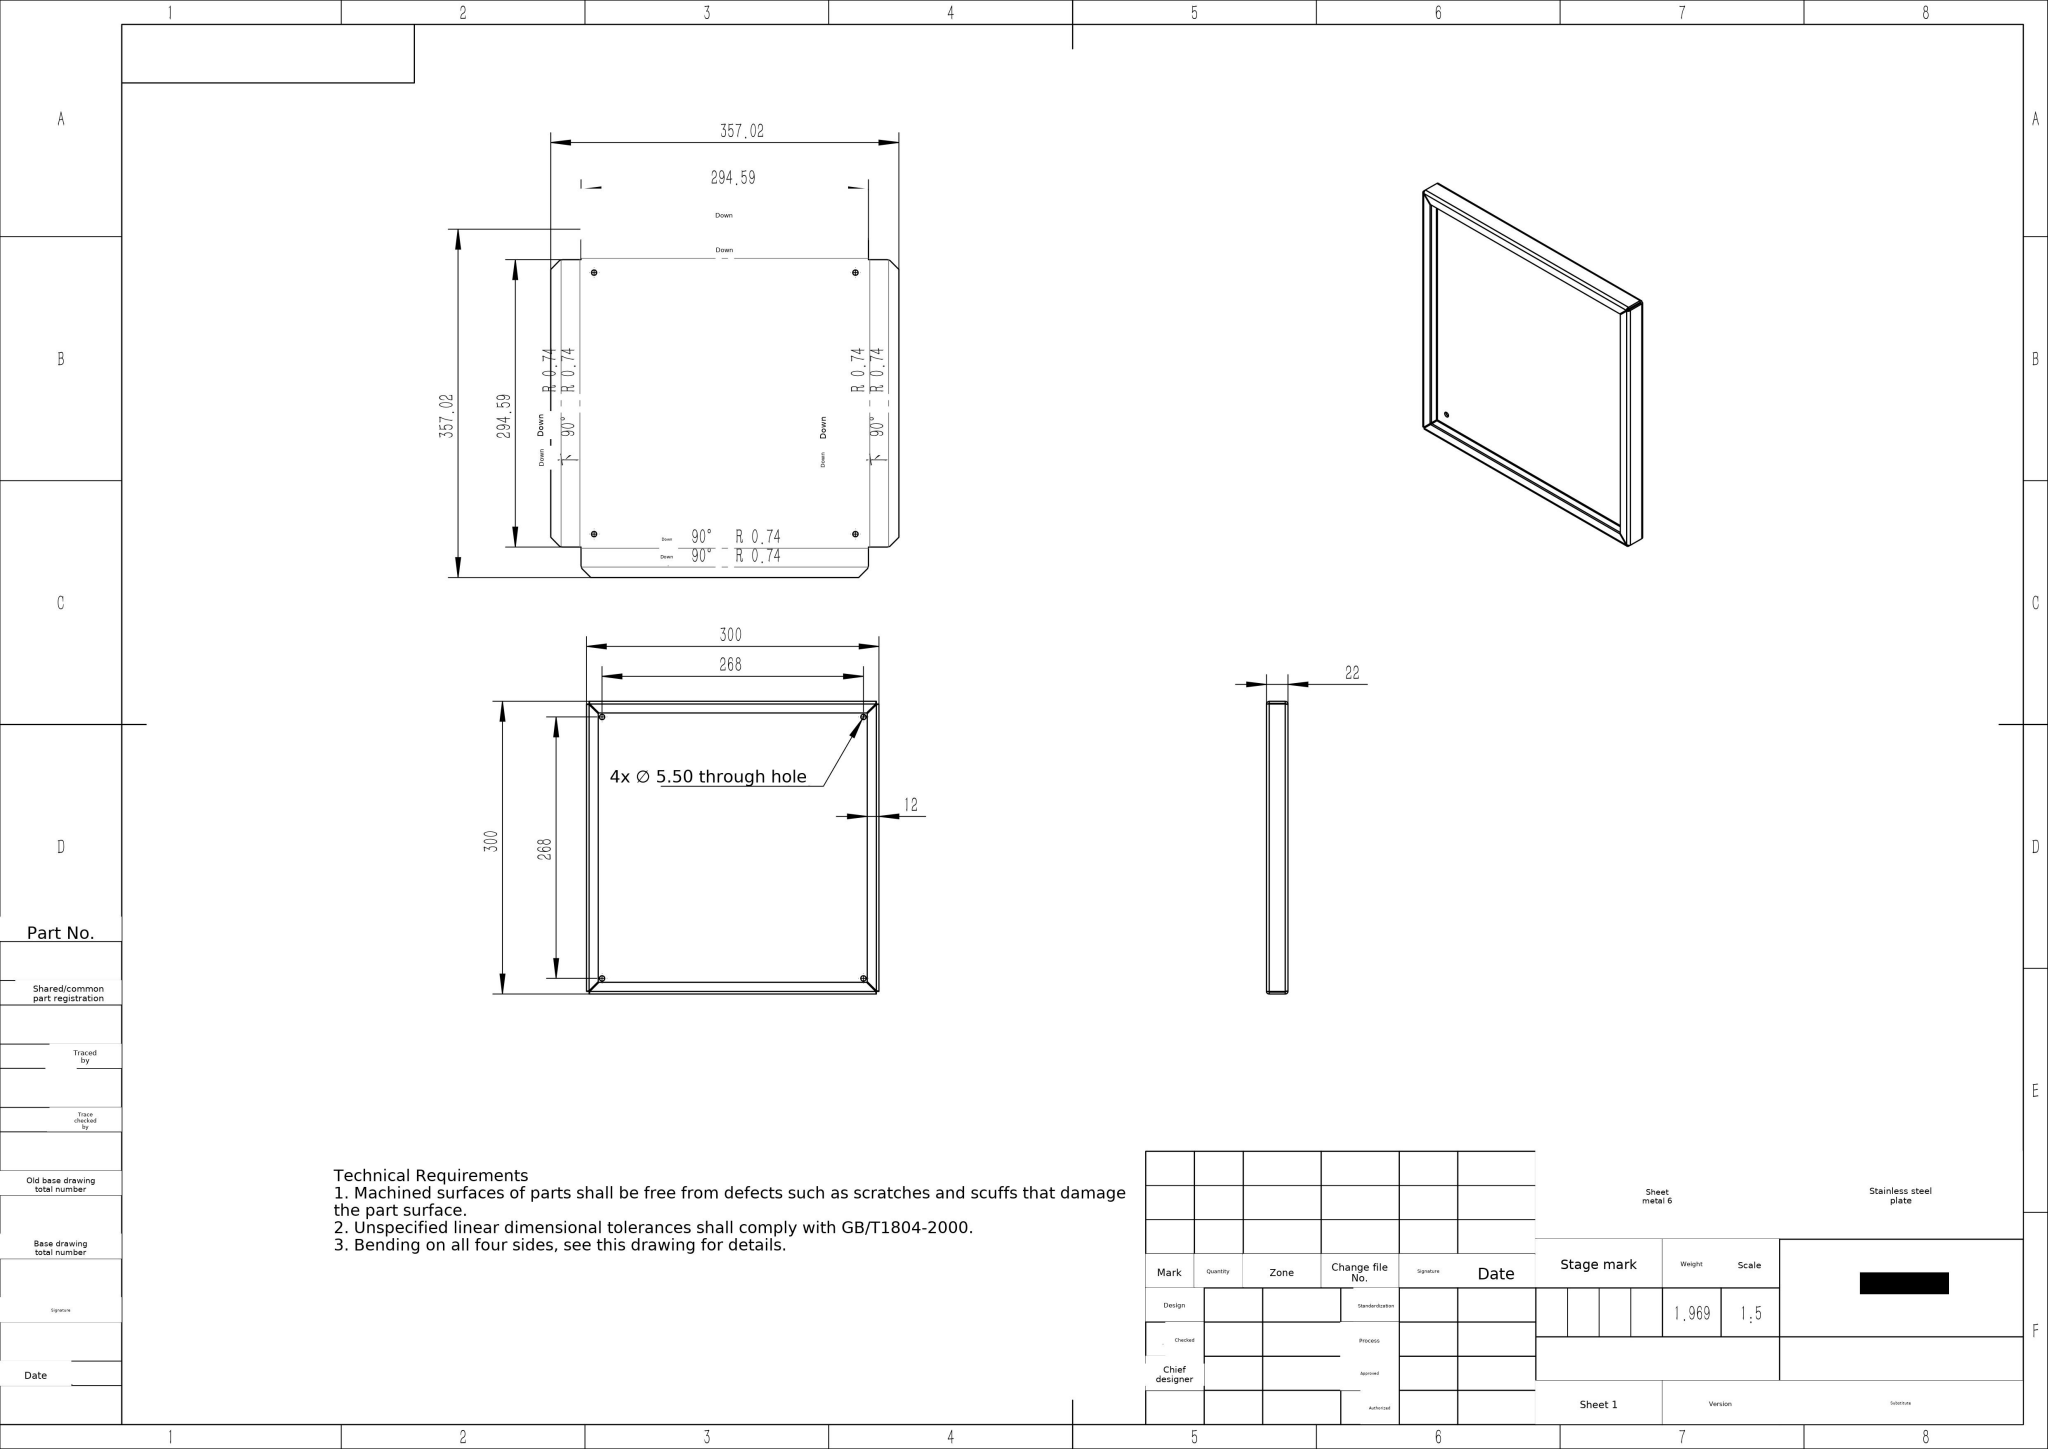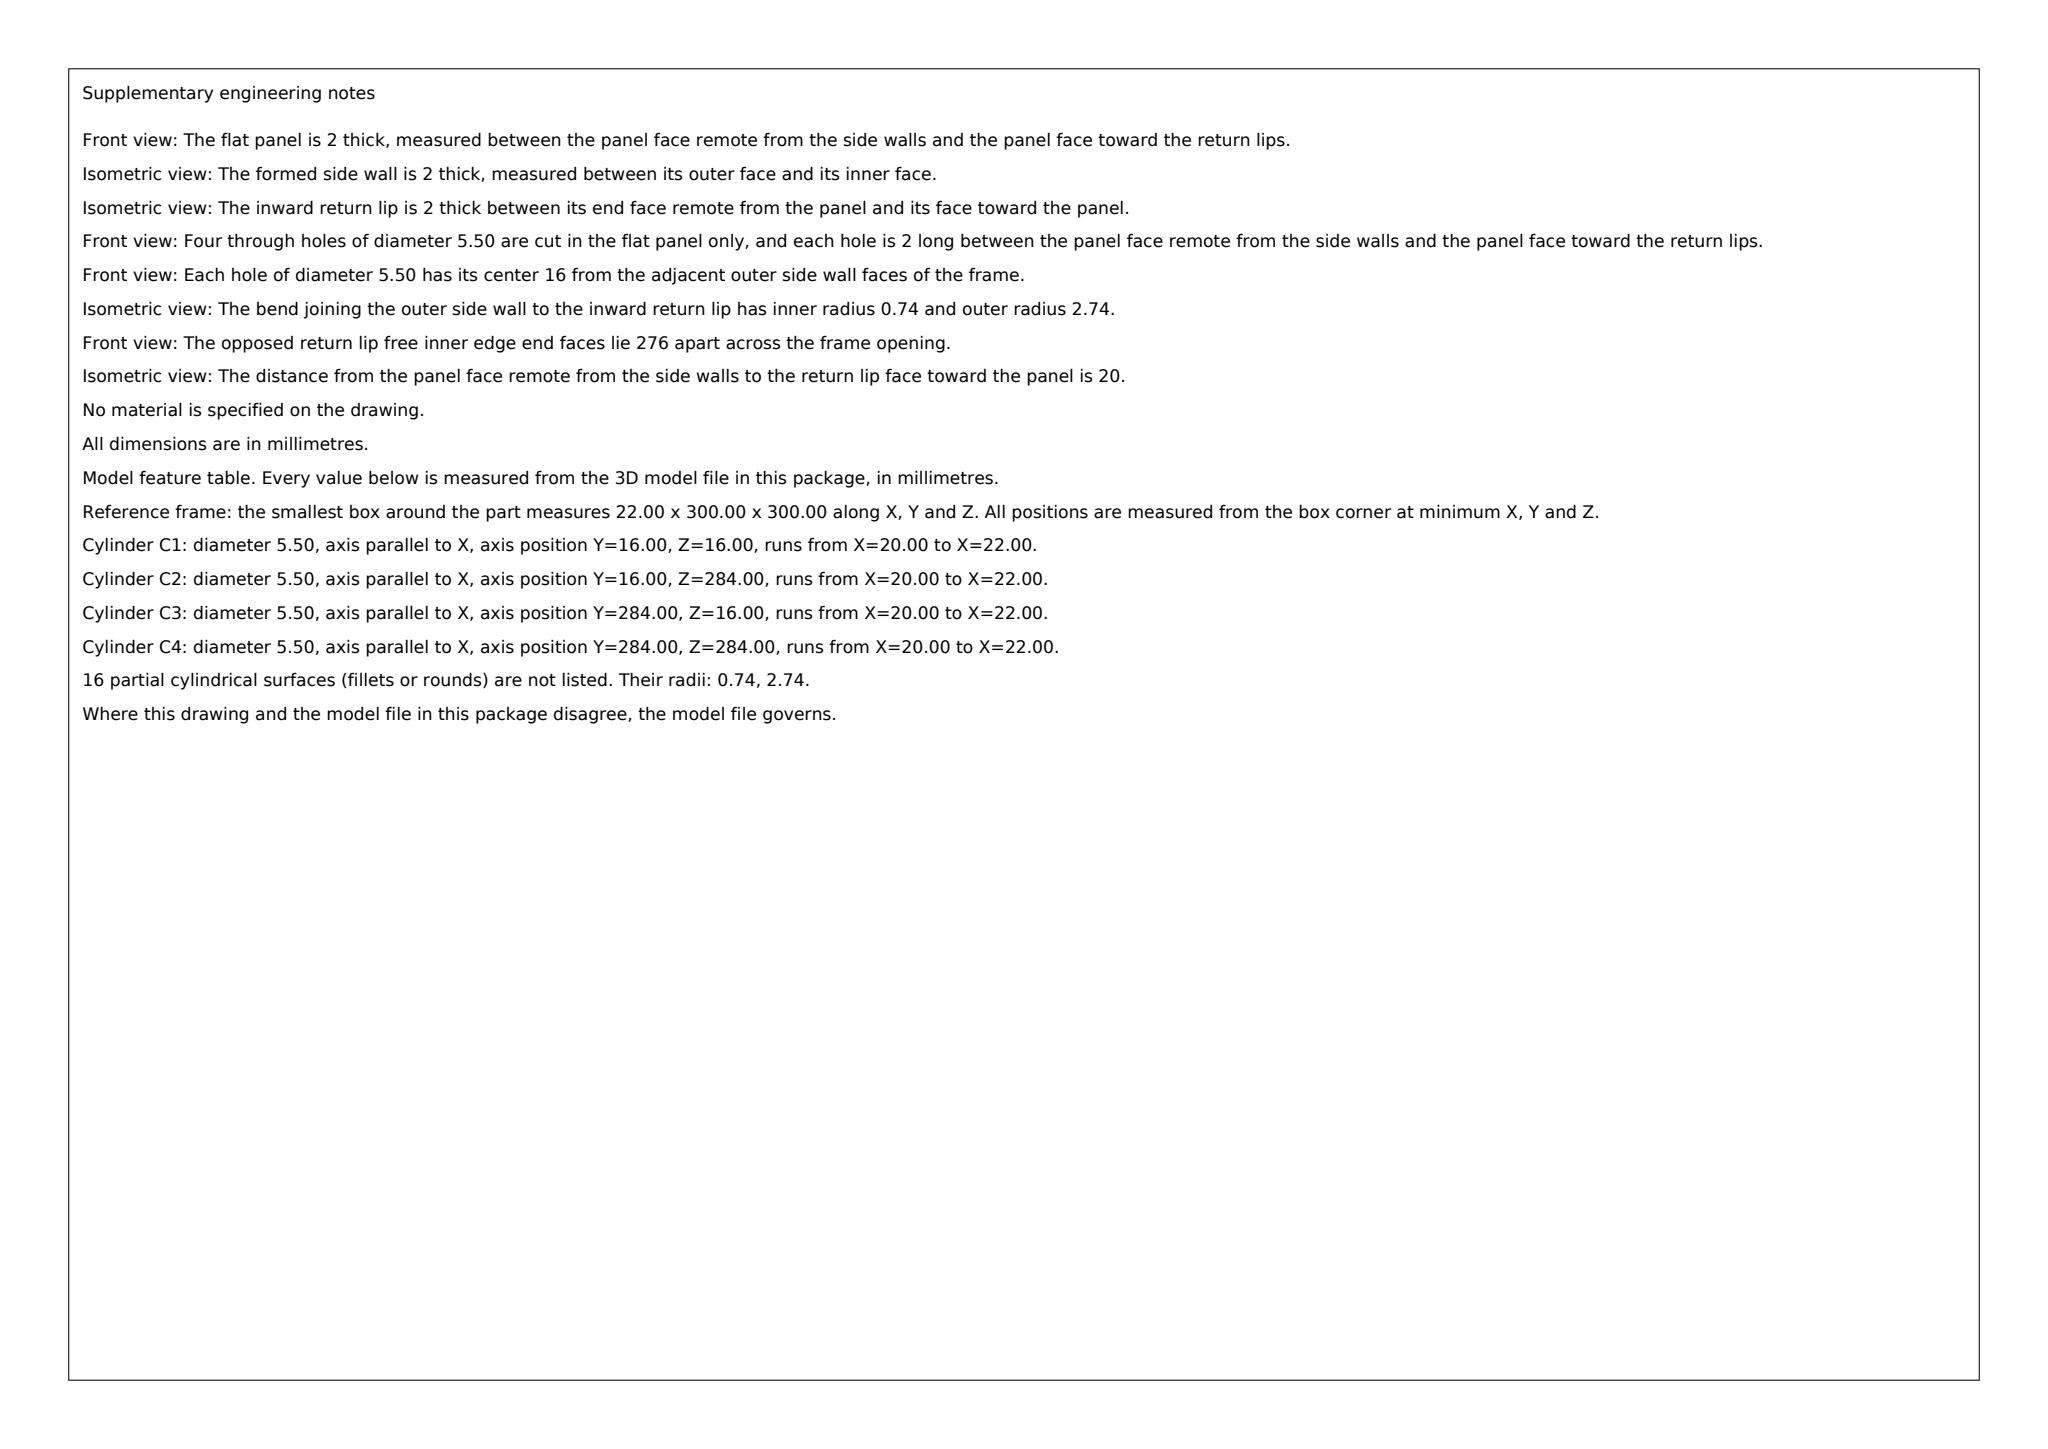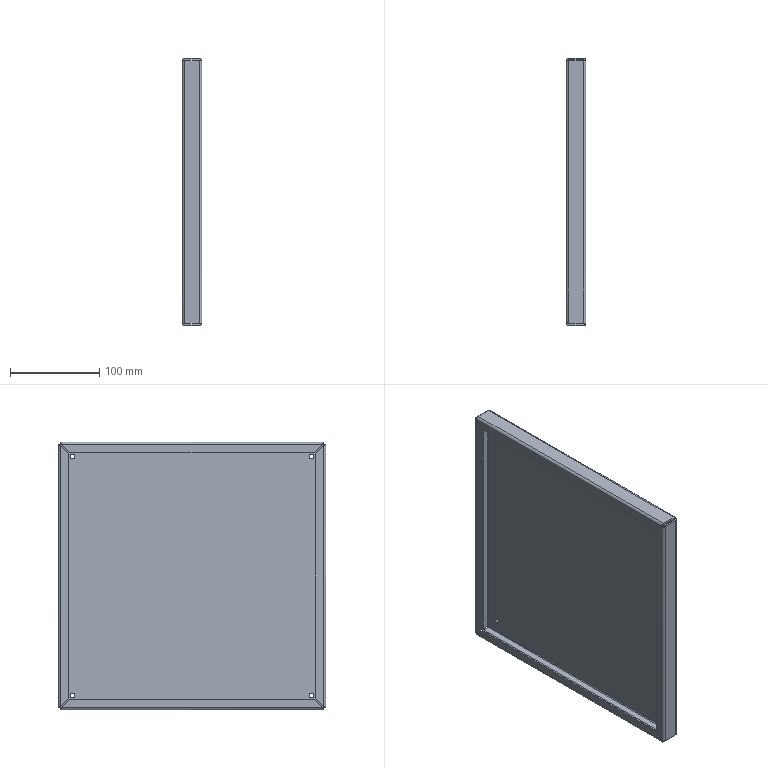Part | SolidWorks | mm | 1 solid | 78 faces | box 22 x 300 x 300 mm | volume 246126 mm3 | plane 38 | cylinder 24 | spline 16 | commonest cylinder face diameters 5.5 x8 5.473 x8 1.473 x8